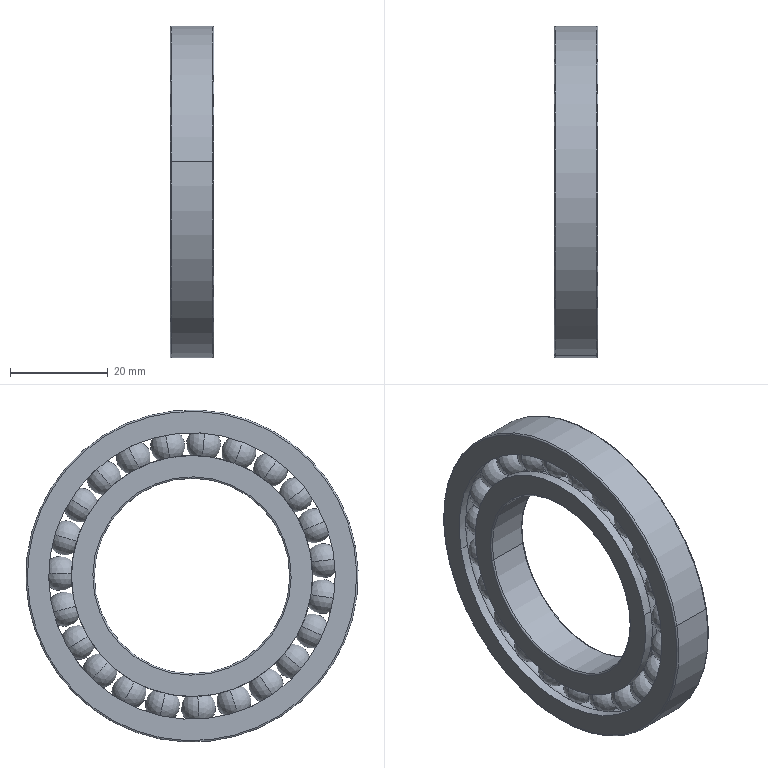Component | SolidWorks | SeedingAssemblyA-1_16008Bearing-2 | 1 solid | 142 faces | volume 16956 mm3 | torus 80 | sphere 46 | cylinder 12 | plane 4 | commonest cylinder face diameters 58.667 x4 49.333 x4 68 x2 40 x2